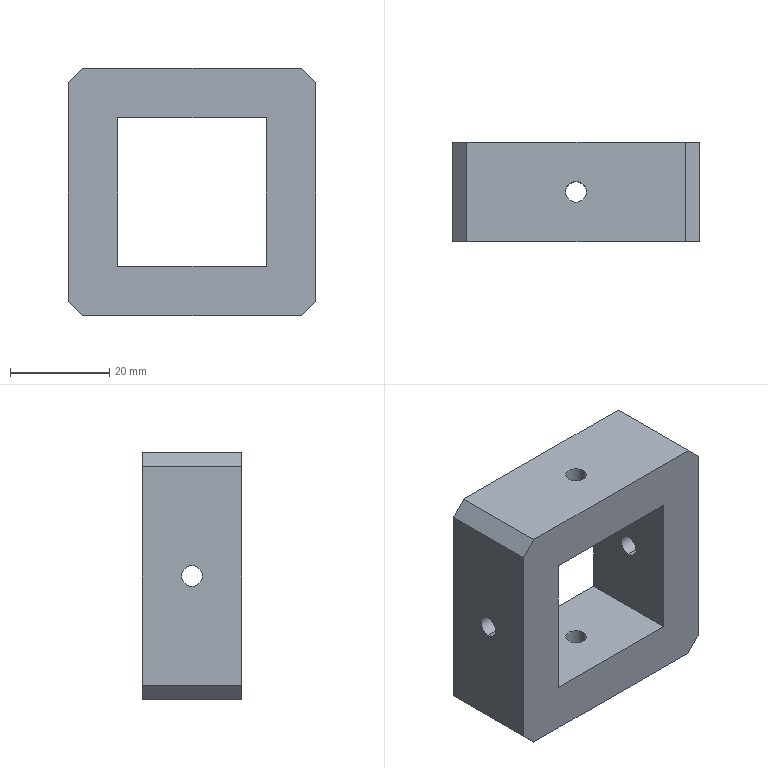Component | SolidWorks | LimitingBlock-1 | 1 solid | 22 faces | box 50 x 20 x 50 mm | volume 31086 mm3 | plane 14 | cylinder 8 | commonest cylinder face diameters 4.2 x8
build123d program:
from build123d import *

# Parameters (mm, degrees)
SKETCH1_W           = 50
SKETCH1_H           = 50
SKETCH1_W_2         = 30
SKETCH1_H_2         = 30
BOSS_EXTRUDE1_DEPTH = 20
CIRPATTERN1_COUNT   = 4
CHAMFER1_SIZE       = 3


with BuildPart() as part:
    # Sketch1 → Boss-Extrude1 (new body)
    with BuildSketch(Plane(origin=(0, 0, 0), x_dir=(1, 0, 0), z_dir=(0, 1, 0))):
        Rectangle(SKETCH1_W, SKETCH1_H)
        Rectangle(SKETCH1_W_2, SKETCH1_H_2, mode=Mode.SUBTRACT)
    extrude(amount=BOSS_EXTRUDE1_DEPTH)

    # Sketch3 → M5 Tapped Hole1 (revolve, cut)
    with BuildSketch(Plane(origin=(0, 10, -25), x_dir=(0, 1, 0), z_dir=(1, 0, 0))):
        Polygon((0, 0), (0, 13.662), (2.1, 12.4), (2.1, 0), align=None)
    m5_tapped_hole1 = revolve(axis=Axis((0, 10, -31.35), (0, 0, 1)), mode=Mode.SUBTRACT)

    # CirPattern1: M5 Tapped Hole1 ×4 about axis
    cirpattern1_axis = Axis((0, 0, 0), (0, 1, 0))
    for i in range(1, CIRPATTERN1_COUNT):
        add(m5_tapped_hole1.rotate(cirpattern1_axis, i * 360 / CIRPATTERN1_COUNT), mode=Mode.SUBTRACT)

    # Chamfer1
    chamfer1_edges = [part.edges().sort_by_distance(p)[0] for p in [
        (-25, 10, -25),
        (25, 10, -25),
        (25, 10, 25),
        (-25, 10, 25),
    ]]
    chamfer(chamfer1_edges, length=CHAMFER1_SIZE)


solid = part.part

# Placed as in the assembly
solid = solid.moved(Location((-29.507, 6.589, 458), (0, 0, 0)))
STEP:
#1=COLOUR_RGB('',0.7922,0.8196,0.9333);
#2=FILL_AREA_STYLE_COLOUR('',#1);
#3=FILL_AREA_STYLE('',(#2));
#4=SURFACE_STYLE_FILL_AREA(#3);
#5=SURFACE_SIDE_STYLE('',(#4));
#6=SURFACE_STYLE_USAGE(.BOTH.,#5);
#7=PRESENTATION_STYLE_ASSIGNMENT((#6));
#8=CARTESIAN_POINT('',(-0.5711,0.6531,17.949));
#9=VERTEX_POINT('',#8);
#10=CARTESIAN_POINT('',(-0.5711,0.6531,18.114));
#11=VERTEX_POINT('',#10);
#12=CARTESIAN_POINT('',(-0.5711,0.6531,18.031));
#13=DIRECTION('',(-1.,0.,0.));
#14=DIRECTION('',(0.,0.,1.));
#15=AXIS2_PLACEMENT_3D('',#12,#13,#14);
#16=CIRCLE('',#15,0.08268);
#17=EDGE_CURVE('',#9,#11,#16,.T.);
#18=ORIENTED_EDGE('',*,*,#17,.T.);
#19=CARTESIAN_POINT('',(-0.1774,0.6531,18.114));
#20=VERTEX_POINT('',#19);
#21=CARTESIAN_POINT('',(-0.1774,0.6531,18.114));
#22=DIRECTION('',(1.,0.,-0.));
#23=VECTOR('',#22,39.37);
#24=LINE('',#21,#23);
#25=EDGE_CURVE('',#11,#20,#24,.T.);
#26=ORIENTED_EDGE('',*,*,#25,.T.);
#27=CARTESIAN_POINT('',(-0.1774,0.6531,17.949));
#28=VERTEX_POINT('',#27);
#29=CARTESIAN_POINT('',(-0.1774,0.6531,18.031));
#30=DIRECTION('',(1.,0.,-0.));
#31=DIRECTION('',(-0.,0.,-1.));
#32=AXIS2_PLACEMENT_3D('',#29,#30,#31);
#33=CIRCLE('',#32,0.08268);
#34=EDGE_CURVE('',#20,#28,#33,.T.);
#35=ORIENTED_EDGE('',*,*,#34,.T.);
#36=CARTESIAN_POINT('',(-0.1774,0.6531,17.949));
#37=DIRECTION('',(1.,0.,-0.));
#38=VECTOR('',#37,39.37);
#39=LINE('',#36,#38);
#40=EDGE_CURVE('',#9,#28,#39,.T.);
#41=ORIENTED_EDGE('',*,*,#40,.F.);
#42=EDGE_LOOP('',(#18,#26,#35,#41));
#43=FACE_OUTER_BOUND('',#42,.T.);
#44=CARTESIAN_POINT('',(-0.1774,0.6531,18.031));
#45=DIRECTION('',(1.,0.,-0.));
#46=DIRECTION('',(-0.,0.,-1.));
#47=AXIS2_PLACEMENT_3D('',#44,#45,#46);
#48=CYLINDRICAL_SURFACE('',#47,0.08268);
#49=ADVANCED_FACE('',(#43),#48,.F.);
#50=CARTESIAN_POINT('',(-1.079,0.6531,18.622));
#51=VERTEX_POINT('',#50);
#52=CARTESIAN_POINT('',(-1.244,0.6531,18.622));
#53=VERTEX_POINT('',#52);
#54=CARTESIAN_POINT('',(-1.162,0.6531,18.622));
#55=DIRECTION('',(0.,0.,-1.));
#56=DIRECTION('',(-1.,0.,0.));
#57=AXIS2_PLACEMENT_3D('',#54,#55,#56);
#58=CIRCLE('',#57,0.08268);
#59=EDGE_CURVE('',#51,#53,#58,.T.);
#60=ORIENTED_EDGE('',*,*,#59,.T.);
#61=CARTESIAN_POINT('',(-1.244,0.6531,19.016));
#62=VERTEX_POINT('',#61);
#63=CARTESIAN_POINT('',(-1.244,0.6531,19.016));
#64=DIRECTION('',(0.,0.,1.));
#65=VECTOR('',#64,39.37);
#66=LINE('',#63,#65);
#67=EDGE_CURVE('',#53,#62,#66,.T.);
#68=ORIENTED_EDGE('',*,*,#67,.T.);
#69=CARTESIAN_POINT('',(-1.079,0.6531,19.016));
#70=VERTEX_POINT('',#69);
#71=CARTESIAN_POINT('',(-1.162,0.6531,19.016));
#72=DIRECTION('',(0.,0.,1.));
#73=DIRECTION('',(1.,0.,0.));
#74=AXIS2_PLACEMENT_3D('',#71,#72,#73);
#75=CIRCLE('',#74,0.08268);
#76=EDGE_CURVE('',#62,#70,#75,.T.);
#77=ORIENTED_EDGE('',*,*,#76,.T.);
#78=CARTESIAN_POINT('',(-1.079,0.6531,19.016));
#79=DIRECTION('',(0.,0.,1.));
#80=VECTOR('',#79,39.37);
#81=LINE('',#78,#80);
#82=EDGE_CURVE('',#51,#70,#81,.T.);
#83=ORIENTED_EDGE('',*,*,#82,.F.);
#84=EDGE_LOOP('',(#60,#68,#77,#83));
#85=FACE_OUTER_BOUND('',#84,.T.);
#86=CARTESIAN_POINT('',(-1.162,0.6531,19.016));
#87=DIRECTION('',(0.,0.,1.));
#88=DIRECTION('',(1.,0.,0.));
#89=AXIS2_PLACEMENT_3D('',#86,#87,#88);
#90=CYLINDRICAL_SURFACE('',#89,0.08268);
#91=ADVANCED_FACE('',(#85),#90,.F.);
#92=CARTESIAN_POINT('',(-1.752,0.6531,18.114));
#93=VERTEX_POINT('',#92);
#94=CARTESIAN_POINT('',(-1.752,0.6531,17.949));
#95=VERTEX_POINT('',#94);
#96=CARTESIAN_POINT('',(-1.752,0.6531,18.031));
#97=DIRECTION('',(1.,0.,-0.));
#98=DIRECTION('',(0.,0.,-1.));
#99=AXIS2_PLACEMENT_3D('',#96,#97,#98);
#100=CIRCLE('',#99,0.08268);
#101=EDGE_CURVE('',#93,#95,#100,.T.);
#102=ORIENTED_EDGE('',*,*,#101,.T.);
#103=CARTESIAN_POINT('',(-2.146,0.6531,17.949));
#104=VERTEX_POINT('',#103);
#105=CARTESIAN_POINT('',(-2.146,0.6531,17.949));
#106=DIRECTION('',(-1.,0.,0.));
#107=VECTOR('',#106,39.37);
#108=LINE('',#105,#107);
#109=EDGE_CURVE('',#95,#104,#108,.T.);
#110=ORIENTED_EDGE('',*,*,#109,.T.);
#111=CARTESIAN_POINT('',(-2.146,0.6531,18.114));
#112=VERTEX_POINT('',#111);
#113=CARTESIAN_POINT('',(-2.146,0.6531,18.031));
#114=DIRECTION('',(-1.,0.,0.));
#115=DIRECTION('',(0.,0.,1.));
#116=AXIS2_PLACEMENT_3D('',#113,#114,#115);
#117=CIRCLE('',#116,0.08268);
#118=EDGE_CURVE('',#104,#112,#117,.T.);
#119=ORIENTED_EDGE('',*,*,#118,.T.);
#120=CARTESIAN_POINT('',(-2.146,0.6531,18.114));
#121=DIRECTION('',(-1.,0.,0.));
#122=VECTOR('',#121,39.37);
#123=LINE('',#120,#122);
#124=EDGE_CURVE('',#93,#112,#123,.T.);
#125=ORIENTED_EDGE('',*,*,#124,.F.);
#126=EDGE_LOOP('',(#102,#110,#119,#125));
#127=FACE_OUTER_BOUND('',#126,.T.);
#128=CARTESIAN_POINT('',(-2.146,0.6531,18.031));
#129=DIRECTION('',(-1.,0.,0.));
#130=DIRECTION('',(0.,0.,1.));
#131=AXIS2_PLACEMENT_3D('',#128,#129,#130);
#132=CYLINDRICAL_SURFACE('',#131,0.08268);
#133=ADVANCED_FACE('',(#127),#132,.F.);
#134=CARTESIAN_POINT('',(-1.244,0.6531,17.441));
#135=VERTEX_POINT('',#134);
#136=CARTESIAN_POINT('',(-1.079,0.6531,17.441));
#137=VERTEX_POINT('',#136);
#138=CARTESIAN_POINT('',(-1.162,0.6531,17.441));
#139=DIRECTION('',(0.,0.,1.));
#140=DIRECTION('',(1.,0.,0.));
#141=AXIS2_PLACEMENT_3D('',#138,#139,#140);
#142=CIRCLE('',#141,0.08268);
#143=EDGE_CURVE('',#135,#137,#142,.T.);
#144=ORIENTED_EDGE('',*,*,#143,.T.);
#145=CARTESIAN_POINT('',(-1.079,0.6531,17.047));
#146=VERTEX_POINT('',#145);
#147=CARTESIAN_POINT('',(-1.079,0.6531,17.047));
#148=DIRECTION('',(0.,0.,-1.));
#149=VECTOR('',#148,39.37);
#150=LINE('',#147,#149);
#151=EDGE_CURVE('',#137,#146,#150,.T.);
#152=ORIENTED_EDGE('',*,*,#151,.T.);
#153=CARTESIAN_POINT('',(-1.244,0.6531,17.047));
#154=VERTEX_POINT('',#153);
#155=CARTESIAN_POINT('',(-1.162,0.6531,17.047));
#156=DIRECTION('',(0.,0.,-1.));
#157=DIRECTION('',(-1.,0.,0.));
#158=AXIS2_PLACEMENT_3D('',#155,#156,#157);
#159=CIRCLE('',#158,0.08268);
#160=EDGE_CURVE('',#146,#154,#159,.T.);
#161=ORIENTED_EDGE('',*,*,#160,.T.);
#162=CARTESIAN_POINT('',(-1.244,0.6531,17.047));
#163=DIRECTION('',(0.,0.,-1.));
#164=VECTOR('',#163,39.37);
#165=LINE('',#162,#164);
#166=EDGE_CURVE('',#135,#154,#165,.T.);
#167=ORIENTED_EDGE('',*,*,#166,.F.);
#168=EDGE_LOOP('',(#144,#152,#161,#167));
#169=FACE_OUTER_BOUND('',#168,.T.);
#170=CARTESIAN_POINT('',(-1.162,0.6531,17.047));
#171=DIRECTION('',(0.,0.,-1.));
#172=DIRECTION('',(-1.,0.,0.));
#173=AXIS2_PLACEMENT_3D('',#170,#171,#172);
#174=CYLINDRICAL_SURFACE('',#173,0.08268);
#175=ADVANCED_FACE('',(#169),#174,.F.);
#176=CARTESIAN_POINT('',(-2.028,1.047,19.016));
#177=VERTEX_POINT('',#176);
#178=CARTESIAN_POINT('',(-0.2955,1.047,19.016));
#179=VERTEX_POINT('',#178);
#180=CARTESIAN_POINT('',(-2.146,1.047,19.016));
#181=DIRECTION('',(1.,0.,0.));
#182=VECTOR('',#181,39.37);
#183=LINE('',#180,#182);
#184=EDGE_CURVE('',#177,#179,#183,.T.);
#185=ORIENTED_EDGE('',*,*,#184,.T.);
#186=CARTESIAN_POINT('',(-0.1774,1.047,18.898));
#187=VERTEX_POINT('',#186);
#188=CARTESIAN_POINT('',(-0.2365,1.047,18.957));
#189=DIRECTION('',(0.7071,0.,-0.7071));
#190=VECTOR('',#189,39.37);
#191=LINE('',#188,#190);
#192=EDGE_CURVE('',#179,#187,#191,.T.);
#193=ORIENTED_EDGE('',*,*,#192,.T.);
#194=CARTESIAN_POINT('',(-0.1774,1.047,17.165));
#195=VERTEX_POINT('',#194);
#196=CARTESIAN_POINT('',(-0.1774,1.047,17.047));
#197=DIRECTION('',(-0.,0.,-1.));
#198=VECTOR('',#197,39.37);
#199=LINE('',#196,#198);
#200=EDGE_CURVE('',#187,#195,#199,.T.);
#201=ORIENTED_EDGE('',*,*,#200,.T.);
#202=CARTESIAN_POINT('',(-0.2955,1.047,17.047));
#203=VERTEX_POINT('',#202);
#204=CARTESIAN_POINT('',(-0.2365,1.047,17.106));
#205=DIRECTION('',(-0.7071,0.,-0.7071));
#206=VECTOR('',#205,39.37);
#207=LINE('',#204,#206);
#208=EDGE_CURVE('',#195,#203,#207,.T.);
#209=ORIENTED_EDGE('',*,*,#208,.T.);
#210=CARTESIAN_POINT('',(-2.028,1.047,17.047));
#211=VERTEX_POINT('',#210);
#212=CARTESIAN_POINT('',(-2.146,1.047,17.047));
#213=DIRECTION('',(-1.,0.,0.));
#214=VECTOR('',#213,39.37);
#215=LINE('',#212,#214);
#216=EDGE_CURVE('',#203,#211,#215,.T.);
#217=ORIENTED_EDGE('',*,*,#216,.T.);
#218=CARTESIAN_POINT('',(-2.146,1.047,17.165));
#219=VERTEX_POINT('',#218);
#220=CARTESIAN_POINT('',(-2.087,1.047,17.106));
#221=DIRECTION('',(-0.7071,0.,0.7071));
#222=VECTOR('',#221,39.37);
#223=LINE('',#220,#222);
#224=EDGE_CURVE('',#211,#219,#223,.T.);
#225=ORIENTED_EDGE('',*,*,#224,.T.);
#226=CARTESIAN_POINT('',(-2.146,1.047,18.898));
#227=VERTEX_POINT('',#226);
#228=CARTESIAN_POINT('',(-2.146,1.047,17.047));
#229=DIRECTION('',(0.,0.,1.));
#230=VECTOR('',#229,39.37);
#231=LINE('',#228,#230);
#232=EDGE_CURVE('',#219,#227,#231,.T.);
#233=ORIENTED_EDGE('',*,*,#232,.T.);
#234=CARTESIAN_POINT('',(-2.087,1.047,18.957));
#235=DIRECTION('',(0.7071,0.,0.7071));
#236=VECTOR('',#235,39.37);
#237=LINE('',#234,#236);
#238=EDGE_CURVE('',#227,#177,#237,.T.);
#239=ORIENTED_EDGE('',*,*,#238,.T.);
#240=EDGE_LOOP('',(#185,#193,#201,#209,#217,#225,#233,#239));
#241=FACE_OUTER_BOUND('',#240,.T.);
#242=CARTESIAN_POINT('',(-0.5711,1.047,17.441));
#243=VERTEX_POINT('',#242);
#244=CARTESIAN_POINT('',(-1.752,1.047,17.441));
#245=VERTEX_POINT('',#244);
#246=CARTESIAN_POINT('',(-1.752,1.047,17.441));
#247=DIRECTION('',(-1.,0.,0.));
#248=VECTOR('',#247,39.37);
#249=LINE('',#246,#248);
#250=EDGE_CURVE('',#243,#245,#249,.T.);
#251=ORIENTED_EDGE('',*,*,#250,.F.);
#252=CARTESIAN_POINT('',(-0.5711,1.047,18.622));
#253=VERTEX_POINT('',#252);
#254=CARTESIAN_POINT('',(-0.5711,1.047,17.441));
#255=DIRECTION('',(0.,0.,-1.));
#256=VECTOR('',#255,39.37);
#257=LINE('',#254,#256);
#258=EDGE_CURVE('',#253,#243,#257,.T.);
#259=ORIENTED_EDGE('',*,*,#258,.F.);
#260=CARTESIAN_POINT('',(-1.752,1.047,18.622));
#261=VERTEX_POINT('',#260);
#262=CARTESIAN_POINT('',(-1.752,1.047,18.622));
#263=DIRECTION('',(1.,0.,0.));
#264=VECTOR('',#263,39.37);
#265=LINE('',#262,#264);
#266=EDGE_CURVE('',#261,#253,#265,.T.);
#267=ORIENTED_EDGE('',*,*,#266,.F.);
#268=CARTESIAN_POINT('',(-1.752,1.047,17.441));
#269=DIRECTION('',(0.,0.,1.));
#270=VECTOR('',#269,39.37);
#271=LINE('',#268,#270);
#272=EDGE_CURVE('',#245,#261,#271,.T.);
#273=ORIENTED_EDGE('',*,*,#272,.F.);
#274=EDGE_LOOP('',(#251,#259,#267,#273));
#275=FACE_BOUND('',#274,.T.);
#276=CARTESIAN_POINT('',(-1.162,1.047,18.031));
#277=DIRECTION('',(0.,1.,0.));
#278=DIRECTION('',(0.,0.,1.));
#279=AXIS2_PLACEMENT_3D('',#276,#277,#278);
#280=PLANE('',#279);
#281=ADVANCED_FACE('',(#241,#275),#280,.T.);
#282=CARTESIAN_POINT('',(-0.1774,0.2594,18.898));
#283=VERTEX_POINT('',#282);
#284=CARTESIAN_POINT('',(-0.1774,0.2594,17.165));
#285=VERTEX_POINT('',#284);
#286=CARTESIAN_POINT('',(-0.1774,0.2594,17.047));
#287=DIRECTION('',(-0.,0.,-1.));
#288=VECTOR('',#287,39.37);
#289=LINE('',#286,#288);
#290=EDGE_CURVE('',#283,#285,#289,.T.);
#291=ORIENTED_EDGE('',*,*,#290,.F.);
#292=CARTESIAN_POINT('',(-0.2955,0.2594,19.016));
#293=VERTEX_POINT('',#292);
#294=CARTESIAN_POINT('',(-0.1774,0.2594,18.898));
#295=DIRECTION('',(-0.7071,0.,0.7071));
#296=VECTOR('',#295,39.37);
#297=LINE('',#294,#296);
#298=EDGE_CURVE('',#283,#293,#297,.T.);
#299=ORIENTED_EDGE('',*,*,#298,.T.);
#300=CARTESIAN_POINT('',(-2.028,0.2594,19.016));
#301=VERTEX_POINT('',#300);
#302=CARTESIAN_POINT('',(-2.146,0.2594,19.016));
#303=DIRECTION('',(1.,0.,0.));
#304=VECTOR('',#303,39.37);
#305=LINE('',#302,#304);
#306=EDGE_CURVE('',#301,#293,#305,.T.);
#307=ORIENTED_EDGE('',*,*,#306,.F.);
#308=CARTESIAN_POINT('',(-2.146,0.2594,18.898));
#309=VERTEX_POINT('',#308);
#310=CARTESIAN_POINT('',(-2.028,0.2594,19.016));
#311=DIRECTION('',(-0.7071,0.,-0.7071));
#312=VECTOR('',#311,39.37);
#313=LINE('',#310,#312);
#314=EDGE_CURVE('',#301,#309,#313,.T.);
#315=ORIENTED_EDGE('',*,*,#314,.T.);
#316=CARTESIAN_POINT('',(-2.146,0.2594,17.165));
#317=VERTEX_POINT('',#316);
#318=CARTESIAN_POINT('',(-2.146,0.2594,17.047));
#319=DIRECTION('',(0.,0.,1.));
#320=VECTOR('',#319,39.37);
#321=LINE('',#318,#320);
#322=EDGE_CURVE('',#317,#309,#321,.T.);
#323=ORIENTED_EDGE('',*,*,#322,.F.);
#324=CARTESIAN_POINT('',(-2.028,0.2594,17.047));
#325=VERTEX_POINT('',#324);
#326=CARTESIAN_POINT('',(-2.146,0.2594,17.165));
#327=DIRECTION('',(0.7071,0.,-0.7071));
#328=VECTOR('',#327,39.37);
#329=LINE('',#326,#328);
#330=EDGE_CURVE('',#317,#325,#329,.T.);
#331=ORIENTED_EDGE('',*,*,#330,.T.);
#332=CARTESIAN_POINT('',(-0.2955,0.2594,17.047));
#333=VERTEX_POINT('',#332);
#334=CARTESIAN_POINT('',(-2.146,0.2594,17.047));
#335=DIRECTION('',(-1.,0.,0.));
#336=VECTOR('',#335,39.37);
#337=LINE('',#334,#336);
#338=EDGE_CURVE('',#333,#325,#337,.T.);
#339=ORIENTED_EDGE('',*,*,#338,.F.);
#340=CARTESIAN_POINT('',(-0.2955,0.2594,17.047));
#341=DIRECTION('',(0.7071,0.,0.7071));
#342=VECTOR('',#341,39.37);
#343=LINE('',#340,#342);
#344=EDGE_CURVE('',#333,#285,#343,.T.);
#345=ORIENTED_EDGE('',*,*,#344,.T.);
#346=EDGE_LOOP('',(#291,#299,#307,#315,#323,#331,#339,#345));
#347=FACE_OUTER_BOUND('',#346,.T.);
#348=CARTESIAN_POINT('',(-0.5711,0.2594,18.622));
#349=VERTEX_POINT('',#348);
#350=CARTESIAN_POINT('',(-0.5711,0.2594,17.441));
#351=VERTEX_POINT('',#350);
#352=CARTESIAN_POINT('',(-0.5711,0.2594,17.441));
#353=DIRECTION('',(0.,0.,-1.));
#354=VECTOR('',#353,39.37);
#355=LINE('',#352,#354);
#356=EDGE_CURVE('',#349,#351,#355,.T.);
#357=ORIENTED_EDGE('',*,*,#356,.T.);
#358=CARTESIAN_POINT('',(-1.752,0.2594,17.441));
#359=VERTEX_POINT('',#358);
#360=CARTESIAN_POINT('',(-1.752,0.2594,17.441));
#361=DIRECTION('',(-1.,0.,0.));
#362=VECTOR('',#361,39.37);
#363=LINE('',#360,#362);
#364=EDGE_CURVE('',#351,#359,#363,.T.);
#365=ORIENTED_EDGE('',*,*,#364,.T.);
#366=CARTESIAN_POINT('',(-1.752,0.2594,18.622));
#367=VERTEX_POINT('',#366);
#368=CARTESIAN_POINT('',(-1.752,0.2594,17.441));
#369=DIRECTION('',(0.,0.,1.));
#370=VECTOR('',#369,39.37);
#371=LINE('',#368,#370);
#372=EDGE_CURVE('',#359,#367,#371,.T.);
#373=ORIENTED_EDGE('',*,*,#372,.T.);
#374=CARTESIAN_POINT('',(-1.752,0.2594,18.622));
#375=DIRECTION('',(1.,0.,0.));
#376=VECTOR('',#375,39.37);
#377=LINE('',#374,#376);
#378=EDGE_CURVE('',#367,#349,#377,.T.);
#379=ORIENTED_EDGE('',*,*,#378,.T.);
#380=EDGE_LOOP('',(#357,#365,#373,#379));
#381=FACE_BOUND('',#380,.T.);
#382=CARTESIAN_POINT('',(-1.162,0.2594,18.031));
#383=DIRECTION('',(0.,1.,0.));
#384=DIRECTION('',(0.,0.,1.));
#385=AXIS2_PLACEMENT_3D('',#382,#383,#384);
#386=PLANE('',#385);
#387=ADVANCED_FACE('',(#347,#381),#386,.F.);
#388=CARTESIAN_POINT('',(-2.146,0.6531,18.031));
#389=DIRECTION('',(-1.,0.,0.));
#390=DIRECTION('',(0.,0.,1.));
#391=AXIS2_PLACEMENT_3D('',#388,#389,#390);
#392=CIRCLE('',#391,0.08268);
#393=EDGE_CURVE('',#112,#104,#392,.T.);
#394=ORIENTED_EDGE('',*,*,#393,.F.);
#395=ORIENTED_EDGE('',*,*,#118,.F.);
#396=EDGE_LOOP('',(#394,#395));
#397=FACE_BOUND('',#396,.T.);
#398=ORIENTED_EDGE('',*,*,#322,.T.);
#399=CARTESIAN_POINT('',(-2.146,1.047,18.898));
#400=DIRECTION('',(0.,1.,0.));
#401=VECTOR('',#400,39.37);
#402=LINE('',#399,#401);
#403=EDGE_CURVE('',#309,#227,#402,.T.);
#404=ORIENTED_EDGE('',*,*,#403,.T.);
#405=ORIENTED_EDGE('',*,*,#232,.F.);
#406=CARTESIAN_POINT('',(-2.146,1.047,17.165));
#407=DIRECTION('',(0.,-1.,0.));
#408=VECTOR('',#407,39.37);
#409=LINE('',#406,#408);
#410=EDGE_CURVE('',#219,#317,#409,.T.);
#411=ORIENTED_EDGE('',*,*,#410,.T.);
#412=EDGE_LOOP('',(#398,#404,#405,#411));
#413=FACE_OUTER_BOUND('',#412,.T.);
#414=CARTESIAN_POINT('',(-2.146,1.047,17.047));
#415=DIRECTION('',(1.,0.,-0.));
#416=DIRECTION('',(-0.,0.,-1.));
#417=AXIS2_PLACEMENT_3D('',#414,#415,#416);
#418=PLANE('',#417);
#419=ADVANCED_FACE('',(#397,#413),#418,.F.);
#420=CARTESIAN_POINT('',(-1.162,0.6531,19.016));
#421=DIRECTION('',(0.,0.,1.));
#422=DIRECTION('',(1.,0.,0.));
#423=AXIS2_PLACEMENT_3D('',#420,#421,#422);
#424=CIRCLE('',#423,0.08268);
#425=EDGE_CURVE('',#70,#62,#424,.T.);
#426=ORIENTED_EDGE('',*,*,#425,.F.);
#427=ORIENTED_EDGE('',*,*,#76,.F.);
#428=EDGE_LOOP('',(#426,#427));
#429=FACE_BOUND('',#428,.T.);
#430=ORIENTED_EDGE('',*,*,#306,.T.);
#431=CARTESIAN_POINT('',(-0.2955,1.047,19.016));
#432=DIRECTION('',(0.,1.,0.));
#433=VECTOR('',#432,39.37);
#434=LINE('',#431,#433);
#435=EDGE_CURVE('',#293,#179,#434,.T.);
#436=ORIENTED_EDGE('',*,*,#435,.T.);
#437=ORIENTED_EDGE('',*,*,#184,.F.);
#438=CARTESIAN_POINT('',(-2.028,1.047,19.016));
#439=DIRECTION('',(0.,-1.,0.));
#440=VECTOR('',#439,39.37);
#441=LINE('',#438,#440);
#442=EDGE_CURVE('',#177,#301,#441,.T.);
#443=ORIENTED_EDGE('',*,*,#442,.T.);
#444=EDGE_LOOP('',(#430,#436,#437,#443));
#445=FACE_OUTER_BOUND('',#444,.T.);
#446=CARTESIAN_POINT('',(-2.146,1.047,19.016));
#447=DIRECTION('',(0.,0.,-1.));
#448=DIRECTION('',(-1.,0.,0.));
#449=AXIS2_PLACEMENT_3D('',#446,#447,#448);
#450=PLANE('',#449);
#451=ADVANCED_FACE('',(#429,#445),#450,.F.);
#452=CARTESIAN_POINT('',(-0.1774,0.6531,18.031));
#453=DIRECTION('',(1.,0.,-0.));
#454=DIRECTION('',(-0.,0.,-1.));
#455=AXIS2_PLACEMENT_3D('',#452,#453,#454);
#456=CIRCLE('',#455,0.08268);
#457=EDGE_CURVE('',#28,#20,#456,.T.);
#458=ORIENTED_EDGE('',*,*,#457,.F.);
#459=ORIENTED_EDGE('',*,*,#34,.F.);
#460=EDGE_LOOP('',(#458,#459));
#461=FACE_BOUND('',#460,.T.);
#462=ORIENTED_EDGE('',*,*,#200,.F.);
#463=CARTESIAN_POINT('',(-0.1774,1.047,18.898));
#464=DIRECTION('',(0.,-1.,0.));
#465=VECTOR('',#464,39.37);
#466=LINE('',#463,#465);
#467=EDGE_CURVE('',#187,#283,#466,.T.);
#468=ORIENTED_EDGE('',*,*,#467,.T.);
#469=ORIENTED_EDGE('',*,*,#290,.T.);
#470=CARTESIAN_POINT('',(-0.1774,1.047,17.165));
#471=DIRECTION('',(0.,1.,0.));
#472=VECTOR('',#471,39.37);
#473=LINE('',#470,#472);
#474=EDGE_CURVE('',#285,#195,#473,.T.);
#475=ORIENTED_EDGE('',*,*,#474,.T.);
#476=EDGE_LOOP('',(#462,#468,#469,#475));
#477=FACE_OUTER_BOUND('',#476,.T.);
#478=CARTESIAN_POINT('',(-0.1774,1.047,17.047));
#479=DIRECTION('',(-1.,0.,0.));
#480=DIRECTION('',(0.,0.,1.));
#481=AXIS2_PLACEMENT_3D('',#478,#479,#480);
#482=PLANE('',#481);
#483=ADVANCED_FACE('',(#461,#477),#482,.F.);
#484=CARTESIAN_POINT('',(-1.162,0.6531,17.047));
#485=DIRECTION('',(0.,0.,-1.));
#486=DIRECTION('',(-1.,0.,0.));
#487=AXIS2_PLACEMENT_3D('',#484,#485,#486);
#488=CIRCLE('',#487,0.08268);
#489=EDGE_CURVE('',#154,#146,#488,.T.);
#490=ORIENTED_EDGE('',*,*,#489,.F.);
#491=ORIENTED_EDGE('',*,*,#160,.F.);
#492=EDGE_LOOP('',(#490,#491));
#493=FACE_BOUND('',#492,.T.);
#494=ORIENTED_EDGE('',*,*,#338,.T.);
#495=CARTESIAN_POINT('',(-2.028,1.047,17.047));
#496=DIRECTION('',(0.,1.,0.));
#497=VECTOR('',#496,39.37);
#498=LINE('',#495,#497);
#499=EDGE_CURVE('',#325,#211,#498,.T.);
#500=ORIENTED_EDGE('',*,*,#499,.T.);
#501=ORIENTED_EDGE('',*,*,#216,.F.);
#502=CARTESIAN_POINT('',(-0.2955,1.047,17.047));
#503=DIRECTION('',(0.,-1.,0.));
#504=VECTOR('',#503,39.37);
#505=LINE('',#502,#504);
#506=EDGE_CURVE('',#203,#333,#505,.T.);
#507=ORIENTED_EDGE('',*,*,#506,.T.);
#508=EDGE_LOOP('',(#494,#500,#501,#507));
#509=FACE_OUTER_BOUND('',#508,.T.);
#510=CARTESIAN_POINT('',(-2.146,1.047,17.047));
#511=DIRECTION('',(0.,0.,1.));
#512=DIRECTION('',(1.,0.,0.));
#513=AXIS2_PLACEMENT_3D('',#510,#511,#512);
#514=PLANE('',#513);
#515=ADVANCED_FACE('',(#493,#509),#514,.F.);
#516=ORIENTED_EDGE('',*,*,#17,.F.);
#517=CARTESIAN_POINT('',(-0.5711,0.6531,18.031));
#518=DIRECTION('',(-1.,0.,0.));
#519=DIRECTION('',(0.,0.,1.));
#520=AXIS2_PLACEMENT_3D('',#517,#518,#519);
#521=CIRCLE('',#520,0.08268);
#522=EDGE_CURVE('',#11,#9,#521,.T.);
#523=ORIENTED_EDGE('',*,*,#522,.F.);
#524=EDGE_LOOP('',(#516,#523));
#525=FACE_BOUND('',#524,.T.);
#526=ORIENTED_EDGE('',*,*,#356,.F.);
#527=CARTESIAN_POINT('',(-0.5711,1.047,18.622));
#528=DIRECTION('',(0.,-1.,0.));
#529=VECTOR('',#528,39.37);
#530=LINE('',#527,#529);
#531=EDGE_CURVE('',#253,#349,#530,.T.);
#532=ORIENTED_EDGE('',*,*,#531,.F.);
#533=ORIENTED_EDGE('',*,*,#258,.T.);
#534=CARTESIAN_POINT('',(-0.5711,1.047,17.441));
#535=DIRECTION('',(0.,-1.,0.));
#536=VECTOR('',#535,39.37);
#537=LINE('',#534,#536);
#538=EDGE_CURVE('',#243,#351,#537,.T.);
#539=ORIENTED_EDGE('',*,*,#538,.T.);
#540=EDGE_LOOP('',(#526,#532,#533,#539));
#541=FACE_OUTER_BOUND('',#540,.T.);
#542=CARTESIAN_POINT('',(-0.5711,1.047,17.441));
#543=DIRECTION('',(-1.,0.,0.));
#544=DIRECTION('',(0.,0.,1.));
#545=AXIS2_PLACEMENT_3D('',#542,#543,#544);
#546=PLANE('',#545);
#547=ADVANCED_FACE('',(#525,#541),#546,.T.);
#548=ORIENTED_EDGE('',*,*,#143,.F.);
#549=CARTESIAN_POINT('',(-1.162,0.6531,17.441));
#550=DIRECTION('',(0.,0.,1.));
#551=DIRECTION('',(1.,0.,0.));
#552=AXIS2_PLACEMENT_3D('',#549,#550,#551);
#553=CIRCLE('',#552,0.08268);
#554=EDGE_CURVE('',#137,#135,#553,.T.);
#555=ORIENTED_EDGE('',*,*,#554,.F.);
#556=EDGE_LOOP('',(#548,#555));
#557=FACE_BOUND('',#556,.T.);
#558=ORIENTED_EDGE('',*,*,#364,.F.);
#559=ORIENTED_EDGE('',*,*,#538,.F.);
#560=ORIENTED_EDGE('',*,*,#250,.T.);
#561=CARTESIAN_POINT('',(-1.752,1.047,17.441));
#562=DIRECTION('',(0.,-1.,0.));
#563=VECTOR('',#562,39.37);
#564=LINE('',#561,#563);
#565=EDGE_CURVE('',#245,#359,#564,.T.);
#566=ORIENTED_EDGE('',*,*,#565,.T.);
#567=EDGE_LOOP('',(#558,#559,#560,#566));
#568=FACE_OUTER_BOUND('',#567,.T.);
#569=CARTESIAN_POINT('',(-1.752,1.047,17.441));
#570=DIRECTION('',(0.,0.,1.));
#571=DIRECTION('',(1.,0.,0.));
#572=AXIS2_PLACEMENT_3D('',#569,#570,#571);
#573=PLANE('',#572);
#574=ADVANCED_FACE('',(#557,#568),#573,.T.);
#575=ORIENTED_EDGE('',*,*,#101,.F.);
#576=CARTESIAN_POINT('',(-1.752,0.6531,18.031));
#577=DIRECTION('',(1.,0.,-0.));
#578=DIRECTION('',(0.,0.,-1.));
#579=AXIS2_PLACEMENT_3D('',#576,#577,#578);
#580=CIRCLE('',#579,0.08268);
#581=EDGE_CURVE('',#95,#93,#580,.T.);
#582=ORIENTED_EDGE('',*,*,#581,.F.);
#583=EDGE_LOOP('',(#575,#582));
#584=FACE_BOUND('',#583,.T.);
#585=ORIENTED_EDGE('',*,*,#372,.F.);
#586=ORIENTED_EDGE('',*,*,#565,.F.);
#587=ORIENTED_EDGE('',*,*,#272,.T.);
#588=CARTESIAN_POINT('',(-1.752,1.047,18.622));
#589=DIRECTION('',(0.,-1.,0.));
#590=VECTOR('',#589,39.37);
#591=LINE('',#588,#590);
#592=EDGE_CURVE('',#261,#367,#591,.T.);
#593=ORIENTED_EDGE('',*,*,#592,.T.);
#594=EDGE_LOOP('',(#585,#586,#587,#593));
#595=FACE_OUTER_BOUND('',#594,.T.);
#596=CARTESIAN_POINT('',(-1.752,1.047,17.441));
#597=DIRECTION('',(1.,0.,-0.));
#598=DIRECTION('',(-0.,0.,-1.));
#599=AXIS2_PLACEMENT_3D('',#596,#597,#598);
#600=PLANE('',#599);
#601=ADVANCED_FACE('',(#584,#595),#600,.T.);
#602=ORIENTED_EDGE('',*,*,#59,.F.);
#603=CARTESIAN_POINT('',(-1.162,0.6531,18.622));
#604=DIRECTION('',(0.,0.,-1.));
#605=DIRECTION('',(-1.,0.,0.));
#606=AXIS2_PLACEMENT_3D('',#603,#604,#605);
#607=CIRCLE('',#606,0.08268);
#608=EDGE_CURVE('',#53,#51,#607,.T.);
#609=ORIENTED_EDGE('',*,*,#608,.F.);
#610=EDGE_LOOP('',(#602,#609));
#611=FACE_BOUND('',#610,.T.);
#612=ORIENTED_EDGE('',*,*,#378,.F.);
#613=ORIENTED_EDGE('',*,*,#592,.F.);
#614=ORIENTED_EDGE('',*,*,#266,.T.);
#615=ORIENTED_EDGE('',*,*,#531,.T.);
#616=EDGE_LOOP('',(#612,#613,#614,#615));
#617=FACE_OUTER_BOUND('',#616,.T.);
#618=CARTESIAN_POINT('',(-1.752,1.047,18.622));
#619=DIRECTION('',(0.,0.,-1.));
#620=DIRECTION('',(-1.,0.,0.));
#621=AXIS2_PLACEMENT_3D('',#618,#619,#620);
#622=PLANE('',#621);
#623=ADVANCED_FACE('',(#611,#617),#622,.T.);
#624=ORIENTED_EDGE('',*,*,#151,.F.);
#625=ORIENTED_EDGE('',*,*,#554,.T.);
#626=ORIENTED_EDGE('',*,*,#166,.T.);
#627=ORIENTED_EDGE('',*,*,#489,.T.);
#628=EDGE_LOOP('',(#624,#625,#626,#627));
#629=FACE_OUTER_BOUND('',#628,.T.);
#630=CARTESIAN_POINT('',(-1.162,0.6531,17.047));
#631=DIRECTION('',(0.,0.,-1.));
#632=DIRECTION('',(-1.,0.,0.));
#633=AXIS2_PLACEMENT_3D('',#630,#631,#632);
#634=CYLINDRICAL_SURFACE('',#633,0.08268);
#635=ADVANCED_FACE('',(#629),#634,.F.);
#636=ORIENTED_EDGE('',*,*,#109,.F.);
#637=ORIENTED_EDGE('',*,*,#581,.T.);
#638=ORIENTED_EDGE('',*,*,#124,.T.);
#639=ORIENTED_EDGE('',*,*,#393,.T.);
#640=EDGE_LOOP('',(#636,#637,#638,#639));
#641=FACE_OUTER_BOUND('',#640,.T.);
#642=CARTESIAN_POINT('',(-2.146,0.6531,18.031));
#643=DIRECTION('',(-1.,0.,0.));
#644=DIRECTION('',(0.,0.,1.));
#645=AXIS2_PLACEMENT_3D('',#642,#643,#644);
#646=CYLINDRICAL_SURFACE('',#645,0.08268);
#647=ADVANCED_FACE('',(#641),#646,.F.);
#648=ORIENTED_EDGE('',*,*,#67,.F.);
#649=ORIENTED_EDGE('',*,*,#608,.T.);
#650=ORIENTED_EDGE('',*,*,#82,.T.);
#651=ORIENTED_EDGE('',*,*,#425,.T.);
#652=EDGE_LOOP('',(#648,#649,#650,#651));
#653=FACE_OUTER_BOUND('',#652,.T.);
#654=CARTESIAN_POINT('',(-1.162,0.6531,19.016));
#655=DIRECTION('',(0.,0.,1.));
#656=DIRECTION('',(1.,0.,0.));
#657=AXIS2_PLACEMENT_3D('',#654,#655,#656);
#658=CYLINDRICAL_SURFACE('',#657,0.08268);
#659=ADVANCED_FACE('',(#653),#658,.F.);
#660=ORIENTED_EDGE('',*,*,#25,.F.);
#661=ORIENTED_EDGE('',*,*,#522,.T.);
#662=ORIENTED_EDGE('',*,*,#40,.T.);
#663=ORIENTED_EDGE('',*,*,#457,.T.);
#664=EDGE_LOOP('',(#660,#661,#662,#663));
#665=FACE_OUTER_BOUND('',#664,.T.);
#666=CARTESIAN_POINT('',(-0.1774,0.6531,18.031));
#667=DIRECTION('',(1.,0.,-0.));
#668=DIRECTION('',(-0.,0.,-1.));
#669=AXIS2_PLACEMENT_3D('',#666,#667,#668);
#670=CYLINDRICAL_SURFACE('',#669,0.08268);
#671=ADVANCED_FACE('',(#665),#670,.F.);
#672=ORIENTED_EDGE('',*,*,#192,.F.);
#673=ORIENTED_EDGE('',*,*,#435,.F.);
#674=ORIENTED_EDGE('',*,*,#298,.F.);
#675=ORIENTED_EDGE('',*,*,#467,.F.);
#676=EDGE_LOOP('',(#672,#673,#674,#675));
#677=FACE_OUTER_BOUND('',#676,.T.);
#678=CARTESIAN_POINT('',(-0.1774,1.047,18.898));
#679=DIRECTION('',(-0.7071,0.,-0.7071));
#680=DIRECTION('',(0.,-1.,0.));
#681=AXIS2_PLACEMENT_3D('',#678,#679,#680);
#682=PLANE('',#681);
#683=ADVANCED_FACE('',(#677),#682,.F.);
#684=ORIENTED_EDGE('',*,*,#238,.F.);
#685=ORIENTED_EDGE('',*,*,#403,.F.);
#686=ORIENTED_EDGE('',*,*,#314,.F.);
#687=ORIENTED_EDGE('',*,*,#442,.F.);
#688=EDGE_LOOP('',(#684,#685,#686,#687));
#689=FACE_OUTER_BOUND('',#688,.T.);
#690=CARTESIAN_POINT('',(-2.028,1.047,19.016));
#691=DIRECTION('',(0.7071,0.,-0.7071));
#692=DIRECTION('',(0.,-1.,0.));
#693=AXIS2_PLACEMENT_3D('',#690,#691,#692);
#694=PLANE('',#693);
#695=ADVANCED_FACE('',(#689),#694,.F.);
#696=ORIENTED_EDGE('',*,*,#224,.F.);
#697=ORIENTED_EDGE('',*,*,#499,.F.);
#698=ORIENTED_EDGE('',*,*,#330,.F.);
#699=ORIENTED_EDGE('',*,*,#410,.F.);
#700=EDGE_LOOP('',(#696,#697,#698,#699));
#701=FACE_OUTER_BOUND('',#700,.T.);
#702=CARTESIAN_POINT('',(-2.146,1.047,17.165));
#703=DIRECTION('',(0.7071,0.,0.7071));
#704=DIRECTION('',(0.,-1.,0.));
#705=AXIS2_PLACEMENT_3D('',#702,#703,#704);
#706=PLANE('',#705);
#707=ADVANCED_FACE('',(#701),#706,.F.);
#708=ORIENTED_EDGE('',*,*,#208,.F.);
#709=ORIENTED_EDGE('',*,*,#474,.F.);
#710=ORIENTED_EDGE('',*,*,#344,.F.);
#711=ORIENTED_EDGE('',*,*,#506,.F.);
#712=EDGE_LOOP('',(#708,#709,#710,#711));
#713=FACE_OUTER_BOUND('',#712,.T.);
#714=CARTESIAN_POINT('',(-0.2955,1.047,17.047));
#715=DIRECTION('',(-0.7071,0.,0.7071));
#716=DIRECTION('',(0.,-1.,0.));
#717=AXIS2_PLACEMENT_3D('',#714,#715,#716);
#718=PLANE('',#717);
#719=ADVANCED_FACE('',(#713),#718,.F.);
#720=CLOSED_SHELL('',(#49,#91,#133,#175,#281,#387,#419,#451,#483,#515,#547,#574,#601,#623,#635,#647,#659,#671,#683,#695,#707,#719));
#721=MANIFOLD_SOLID_BREP('',#720);
#722=STYLED_ITEM('',(#7),#721);
#723=(LENGTH_UNIT()NAMED_UNIT(*)SI_UNIT($,.METRE.));
#724=LENGTH_MEASURE_WITH_UNIT(LENGTH_MEASURE(0.0254),#723);
#725=DIMENSIONAL_EXPONENTS(1.,0.,0.,0.,0.,0.,0.);
#726=(CONVERSION_BASED_UNIT('',#724)LENGTH_UNIT()NAMED_UNIT(#725));
#727=UNCERTAINTY_MEASURE_WITH_UNIT(LENGTH_MEASURE(0.00001),#726,'','');
#728=(NAMED_UNIT(*)PLANE_ANGLE_UNIT()SI_UNIT($,.RADIAN.));
#729=(NAMED_UNIT(*)SI_UNIT($,.STERADIAN.)SOLID_ANGLE_UNIT());
#730=(GEOMETRIC_REPRESENTATION_CONTEXT(3)GLOBAL_UNCERTAINTY_ASSIGNED_CONTEXT((#727))GLOBAL_UNIT_ASSIGNED_CONTEXT((#726,#728,#729))REPRESENTATION_CONTEXT('',''));
#731=MECHANICAL_DESIGN_GEOMETRIC_PRESENTATION_REPRESENTATION('',(#722),#730);
#732=PRESENTATION_LAYER_ASSIGNMENT('','',(#722));
#733=CARTESIAN_POINT('',(0.,0.,0.));
#734=DIRECTION('',(0.,0.,1.));
#735=DIRECTION('',(1.,0.,0.));
#736=AXIS2_PLACEMENT_3D('',#733,#734,#735);
#737=(LENGTH_UNIT()NAMED_UNIT(*)SI_UNIT($,.METRE.));
#738=LENGTH_MEASURE_WITH_UNIT(LENGTH_MEASURE(0.0254),#737);
#739=DIMENSIONAL_EXPONENTS(1.,0.,0.,0.,0.,0.,0.);
#740=(CONVERSION_BASED_UNIT('',#738)LENGTH_UNIT()NAMED_UNIT(#739));
#741=UNCERTAINTY_MEASURE_WITH_UNIT(LENGTH_MEASURE(0.00001),#740,'','');
#742=(NAMED_UNIT(*)PLANE_ANGLE_UNIT()SI_UNIT($,.RADIAN.));
#743=(NAMED_UNIT(*)SI_UNIT($,.STERADIAN.)SOLID_ANGLE_UNIT());
#744=(GEOMETRIC_REPRESENTATION_CONTEXT(3)GLOBAL_UNCERTAINTY_ASSIGNED_CONTEXT((#741))GLOBAL_UNIT_ASSIGNED_CONTEXT((#740,#742,#743))REPRESENTATION_CONTEXT('',''));
#745=ADVANCED_BREP_SHAPE_REPRESENTATION('',(#721,#736),#744);